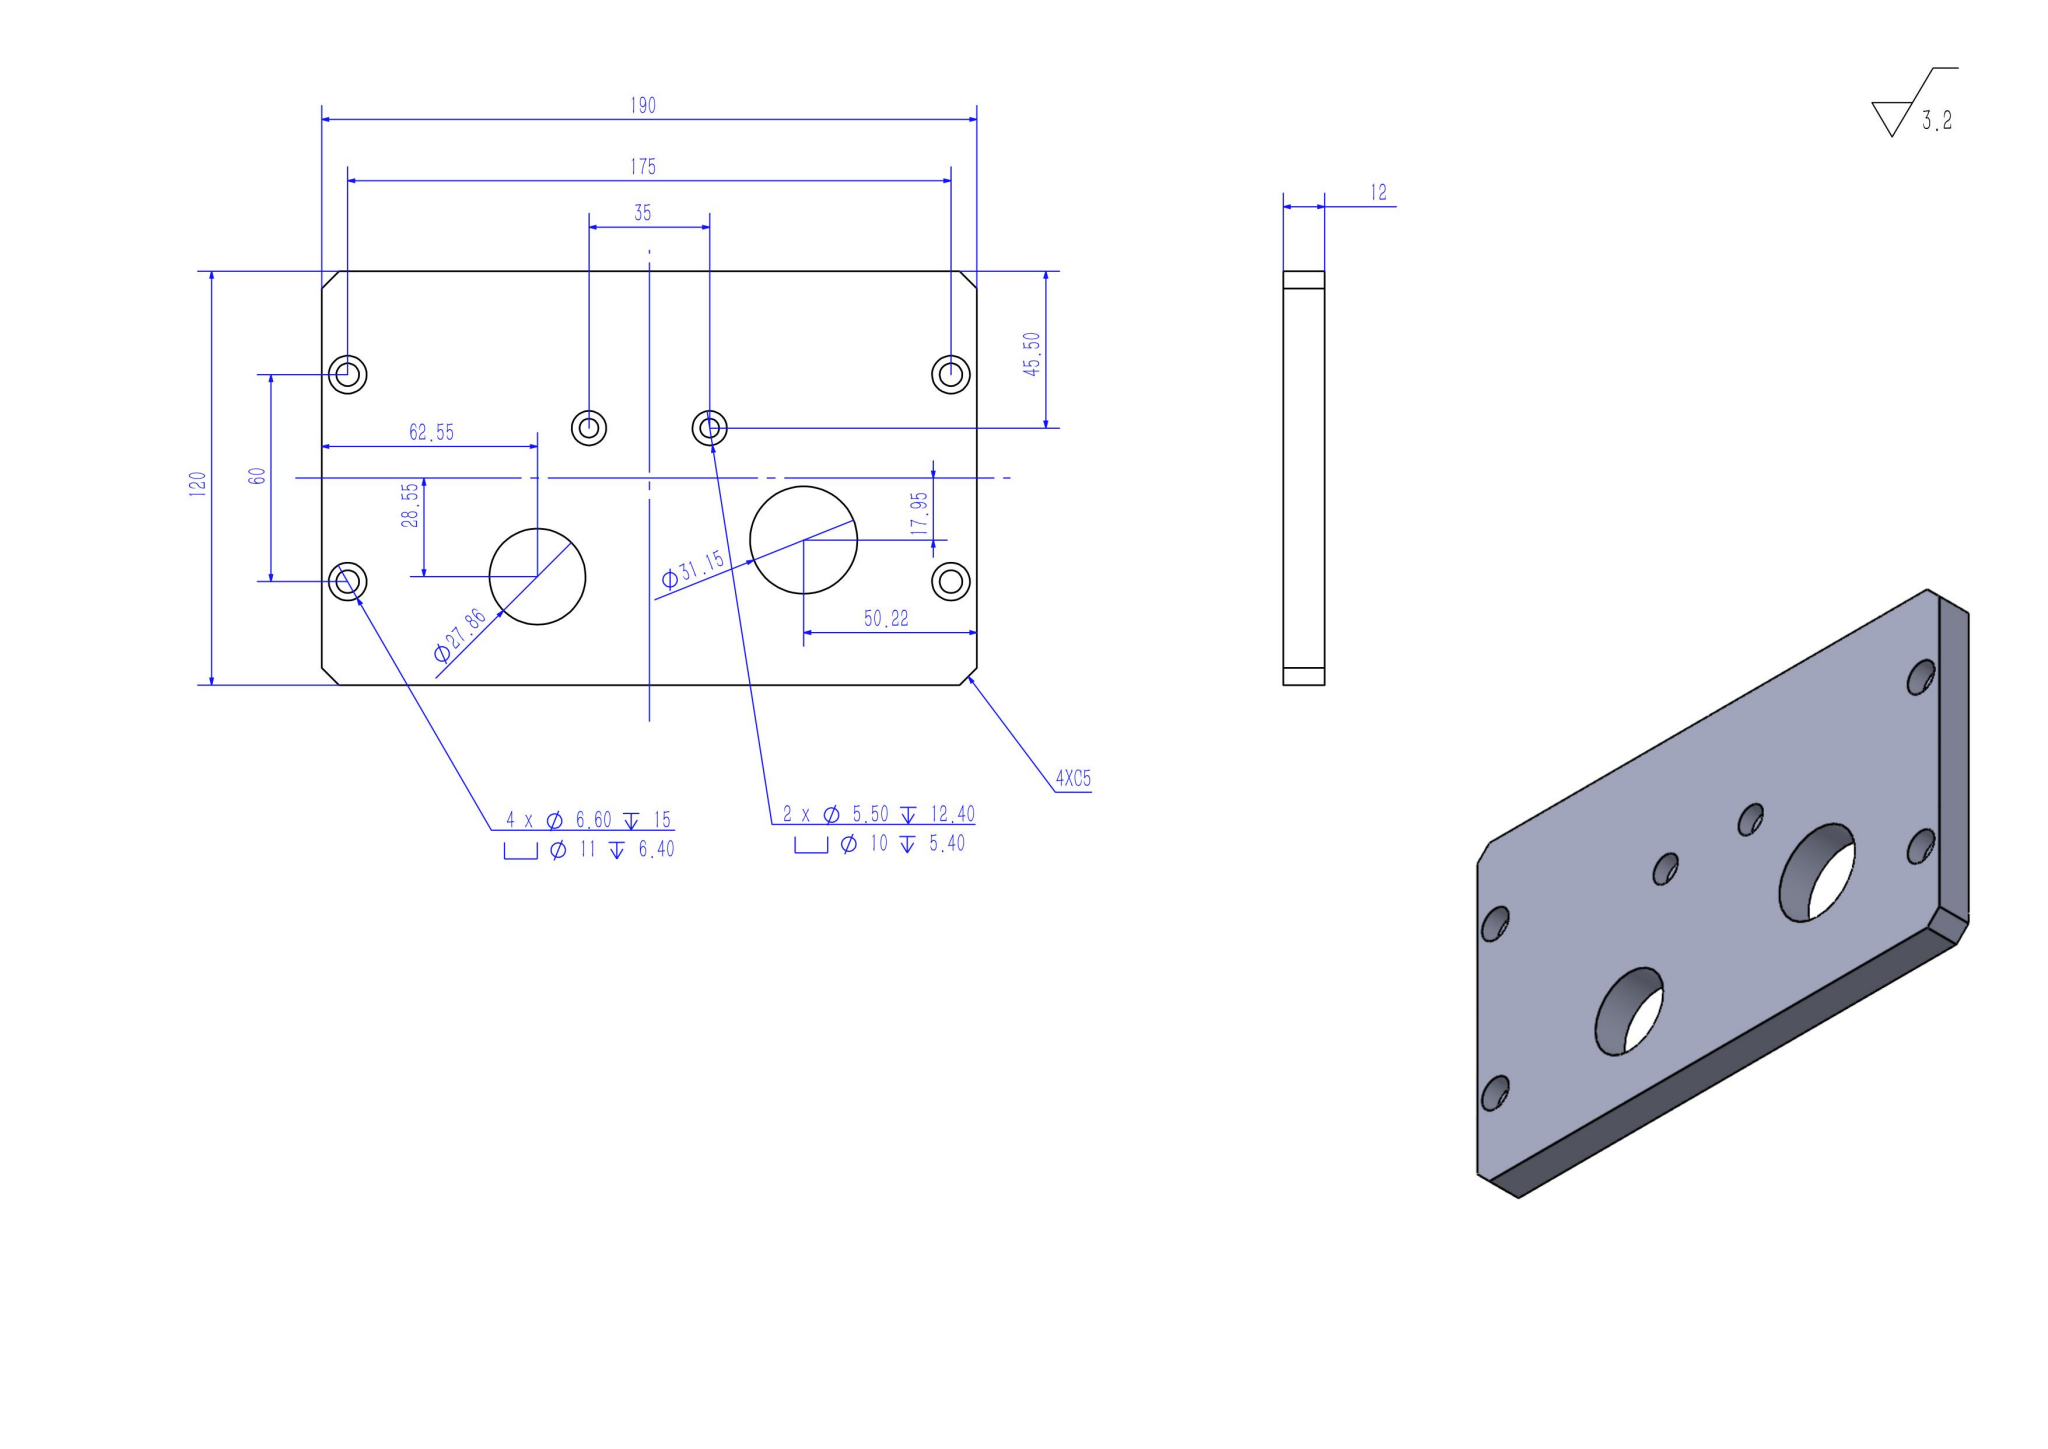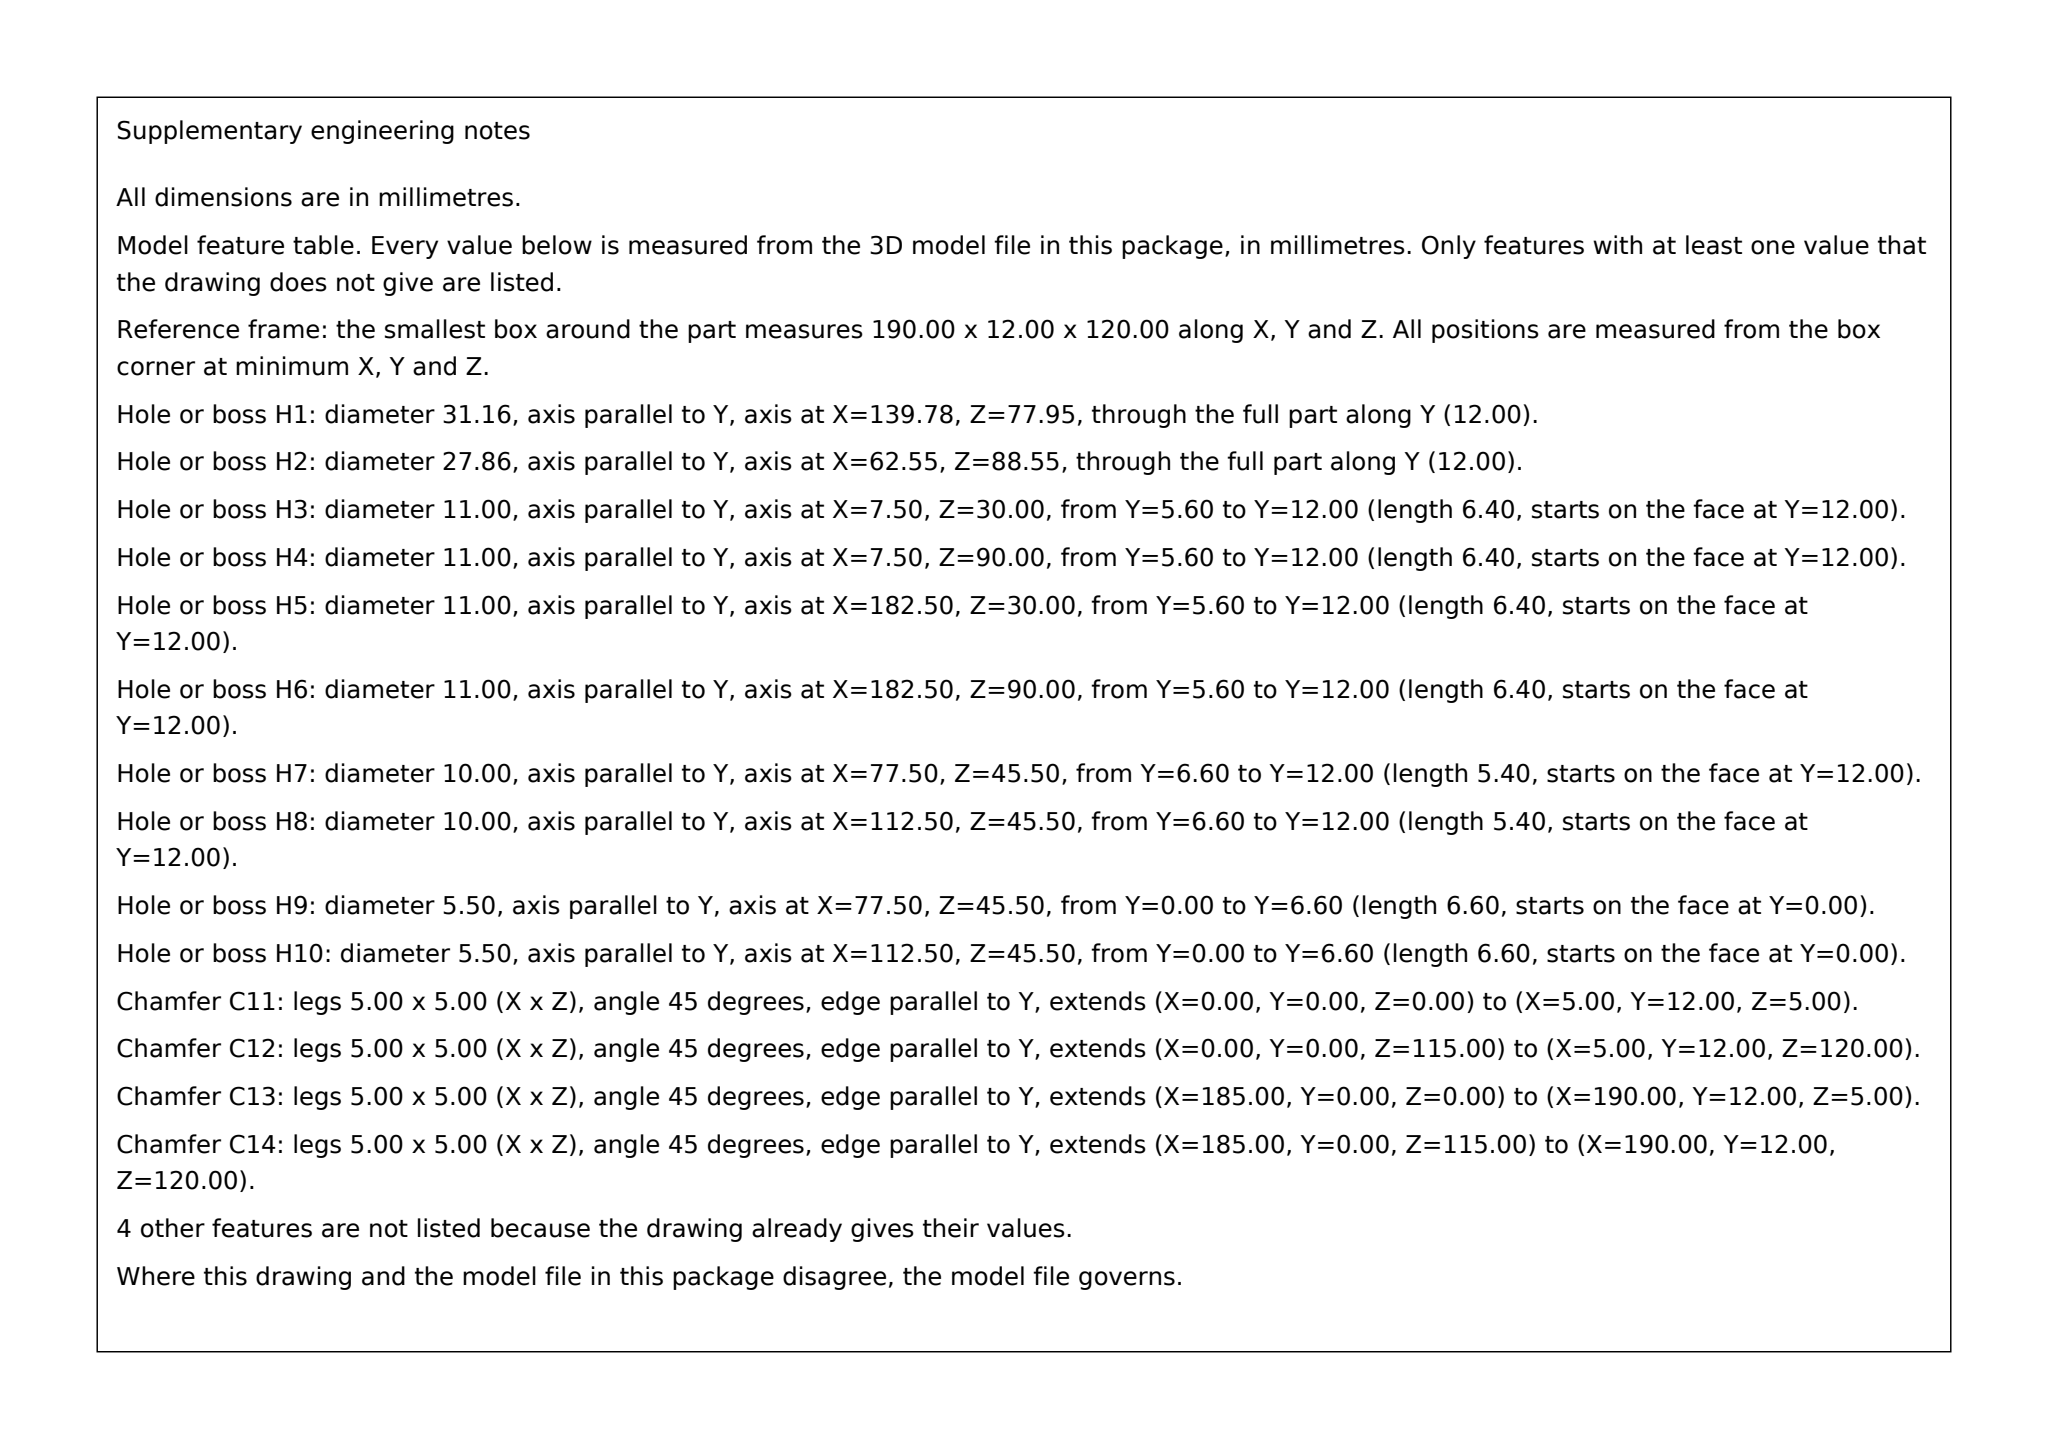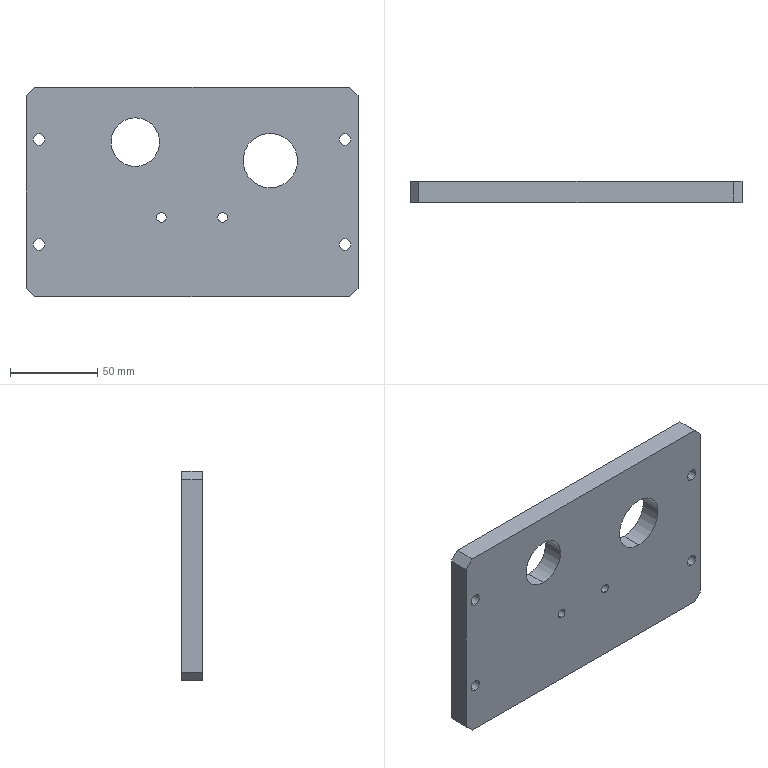Part | SolidWorks | mm | 1 solid | 44 faces | box 190 x 12 x 120 mm | volume 252176 mm3 | cylinder 28 | plane 16 | commonest cylinder face diameters 11 x8 6.6 x8 10 x4 5.5 x4 27.865 x2 31.151 x2
build123d program:
from build123d import *

# Parameters (mm, degrees)
SKETCH1_W                                       = 190
SKETCH1_H                                       = 120
BOSS_EXTRUDE1_DEPTH                             = 12
M6_HEX_SOCKET_HEAD_CAP_SCREW_CBORE1_AT_2_COUNT  = 2
M6_HEX_SOCKET_HEAD_CAP_SCREW_CBORE1_AT_2_PITCH  = 60
CHAMFER1_SIZE                                   = 5
M5_HEX_SOCKET_HEAD_CAP_SCREW_CBORE1_D           = 5.5
M5_HEX_SOCKET_HEAD_CAP_SCREW_CBORE1_DEPTH       = 12.4
M5_HEX_SOCKET_HEAD_CAP_SCREW_CBORE1_CBORE_D     = 10
M5_HEX_SOCKET_HEAD_CAP_SCREW_CBORE1_CBORE_DEPTH = 5.4
M5_HEX_SOCKET_HEAD_CAP_SCREW_CBORE1_TIP         = 1.652
SKETCH8_R                                       = 13.932
SKETCH8_R_2                                     = 15.575
CUT_EXTRUDE1_DEPTH                              = 80


with BuildPart() as part:
    # Sketch1 → Boss-Extrude1 (new body)
    with BuildSketch(Plane(origin=(0, 0, 0), x_dir=(1, 0, 0), z_dir=(0, 1, 0))):
        Rectangle(SKETCH1_W, SKETCH1_H)
    extrude(amount=BOSS_EXTRUDE1_DEPTH)

    # Sketch3 → M6 Hex Socket Head Cap Screw CBORE1 (revolve, cut)
    with BuildSketch(Plane(origin=(87.5, 12, 30), x_dir=(0, 0, 1), z_dir=(1, 0, 0))):
        Polygon((0, 0), (0, 16.983), (3.3, 15), (3.3, 6.4), (5.5, 6.4), (5.5, 0), align=None)
    m6_hex_socket_head_cap_screw_cbore1 = revolve(axis=Axis((87.5, 18.35, 30), (0, -1, 0)), mode=Mode.SUBTRACT)

    # M6 Hex Socket Head Cap Screw CBORE1 at 2: M6 Hex Socket Head Cap Screw CBORE1 ×2
    with Locations(*[(0, 0, -i * M6_HEX_SOCKET_HEAD_CAP_SCREW_CBORE1_AT_2_PITCH) for i in range(1, M6_HEX_SOCKET_HEAD_CAP_SCREW_CBORE1_AT_2_COUNT)]):
        add(m6_hex_socket_head_cap_screw_cbore1, mode=Mode.SUBTRACT)

    # Mirror1: M6 Hex Socket Head Cap Screw CBORE1 across plane
    add(m6_hex_socket_head_cap_screw_cbore1.mirror(Plane(origin=(0, 0, 0), x_dir=(0, 0, 1), z_dir=(1, 0, 0))), mode=Mode.SUBTRACT)

    # Mirror1 copy 1 sketch → Mirror1 copy 1 (revolve, cut)
    with BuildSketch(Plane(origin=(-87.5, 12, -30), x_dir=(0, 0, 1), z_dir=(-1, 0, 0))):
        Polygon((0, 0), (0, -16.983), (3.3, -15), (3.3, -6.4), (5.5, -6.4), (5.5, 0), align=None)
    revolve(axis=Axis((-87.5, 18.35, -30), (0, 1, 0)), mode=Mode.SUBTRACT)

    # Chamfer1
    chamfer1_edges = [part.edges().sort_by_distance(p)[0] for p in [
        (95, 6, 60),
        (-95, 6, 60),
        (-95, 6, -60),
        (95, 6, -60),
    ]]
    chamfer(chamfer1_edges, length=CHAMFER1_SIZE)

    # M5 Hex Socket Head Cap Screw CBORE1
    with Locations(Plane(origin=(0, 12, 0), x_dir=(1, 0, 0), z_dir=(0, 1, 0))):
        with Locations((-17.5, 14.5), (17.5, 14.5)):
            CounterBoreHole(M5_HEX_SOCKET_HEAD_CAP_SCREW_CBORE1_D / 2, M5_HEX_SOCKET_HEAD_CAP_SCREW_CBORE1_CBORE_D / 2, M5_HEX_SOCKET_HEAD_CAP_SCREW_CBORE1_CBORE_DEPTH, depth=M5_HEX_SOCKET_HEAD_CAP_SCREW_CBORE1_DEPTH)
            with Locations((0, 0, -(M5_HEX_SOCKET_HEAD_CAP_SCREW_CBORE1_DEPTH + M5_HEX_SOCKET_HEAD_CAP_SCREW_CBORE1_TIP / 2))):  # 118° drill point
                Cone(0, M5_HEX_SOCKET_HEAD_CAP_SCREW_CBORE1_D / 2, M5_HEX_SOCKET_HEAD_CAP_SCREW_CBORE1_TIP, mode=Mode.SUBTRACT)

    # Sketch8 → Cut-Extrude1 (cut)
    with BuildSketch(Plane(origin=(0, 12, 0), x_dir=(1, 0, 0), z_dir=(0, 1, 0))):
        with Locations(Location((-32.449, -28.555, 0), (0, 0, 270))):
            Circle(SKETCH8_R)
        with Locations(Location((44.779, -17.955, 0), (0, 0, 270))):
            Circle(SKETCH8_R_2)
    extrude(amount=-CUT_EXTRUDE1_DEPTH, mode=Mode.SUBTRACT)


solid = part.part